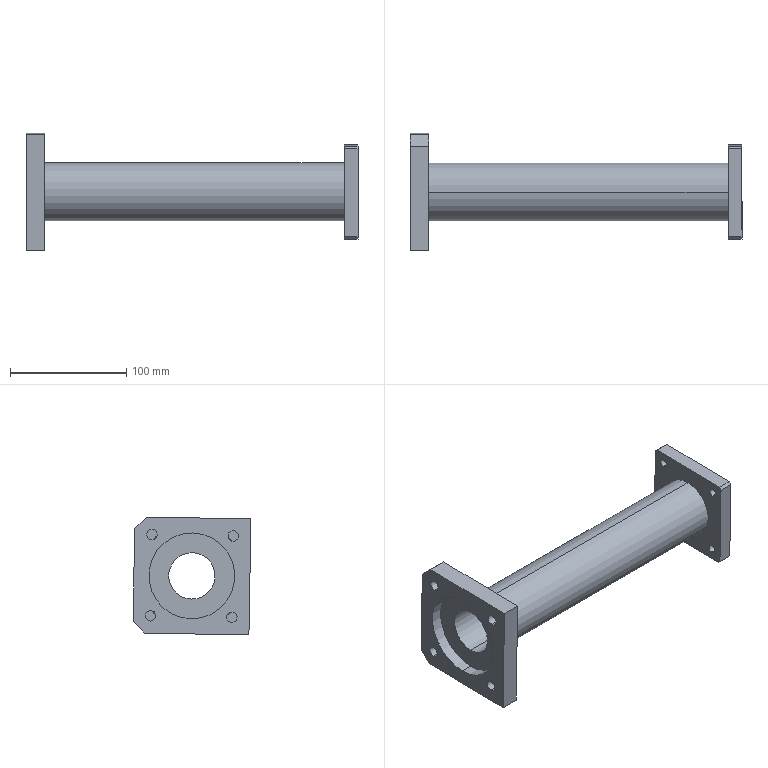Component | SolidWorks | CylinderSeat-1 | 1 solid | 41 faces | box 286 x 101.56 x 101.56 mm | volume 346031 mm3 | cylinder 22 | plane 19 | commonest cylinder face diameters 6.8 x8 9 x8 50 x2 40 x2 74 x2
build123d program:
from build123d import *

# Parameters (mm, degrees)
SKETCH1_W           = 100
SKETCH1_H           = 100
BOSS_EXTRUDE1_DEPTH = 16
SKETCH2_R           = 37
CUT_EXTRUDE1_DEPTH  = 10
SKETCH3_R           = 20
CUT_EXTRUDE2_DEPTH  = 72.414
SKETCH4_R           = 25
SKETCH4_R_2         = 20
BOSS_EXTRUDE2_DEPTH = 258
SKETCH5_W           = 80
SKETCH5_H           = 80
SKETCH5_R           = 20
BOSS_EXTRUDE3_DEPTH = 12
CHAMFER1_SIZE       = 10
SKETCH6_R           = 4.5
CUT_EXTRUDE3_DEPTH  = 20
SKETCH7_R           = 3.4
CUT_EXTRUDE4_DEPTH  = 20
CHAMFER2_SIZE       = 2


with BuildPart() as part:
    # Sketch1 → Boss-Extrude1 (new body)
    with BuildSketch(Plane.XY):
        Rectangle(SKETCH1_W, SKETCH1_H)
    extrude(amount=BOSS_EXTRUDE1_DEPTH)

    # Sketch2 → Cut-Extrude1 (cut)
    with BuildSketch(Plane.XY.offset(16)):
        Circle(SKETCH2_R)
    extrude(amount=-CUT_EXTRUDE1_DEPTH, mode=Mode.SUBTRACT)

    # Sketch3 → Cut-Extrude2 (cut, through all)
    with BuildSketch(Plane.XY.offset(6)):
        Circle(SKETCH3_R)
    extrude(amount=-CUT_EXTRUDE2_DEPTH, mode=Mode.SUBTRACT)

    # Sketch4 → Boss-Extrude2 (add)
    with BuildSketch(Plane(origin=(0, 0, 0), x_dir=(-1, 0, 0), z_dir=(0, 0, -1))):
        with Locations(Location((0, 0, 0), (0, 0, 180))):
            Circle(SKETCH4_R)
        with Locations(Location((0, 0, 0), (0, 0, 180))):
            Circle(SKETCH4_R_2, mode=Mode.SUBTRACT)
    extrude(amount=BOSS_EXTRUDE2_DEPTH)

    # Sketch5 → Boss-Extrude3 (add)
    with BuildSketch(Plane(origin=(0, 0, -258), x_dir=(-1, 0, 0), z_dir=(0, 0, -1))):
        Rectangle(SKETCH5_W, SKETCH5_H)
        with Locations(Location((0, 0, 0), (0, 0, 180))):
            Circle(SKETCH5_R, mode=Mode.SUBTRACT)
    extrude(amount=BOSS_EXTRUDE3_DEPTH)

    # Chamfer1
    chamfer1_edges = [part.edges().sort_by_distance(p)[0] for p in [
        (-50, 50, 8),
        (50, 50, 8),
    ]]
    chamfer(chamfer1_edges, length=CHAMFER1_SIZE)

    # Sketch6 → Cut-Extrude3 (cut)
    with BuildSketch(Plane.XY.offset(16)):
        with Locations((-35, 35)):
            Circle(SKETCH6_R)
        with Locations((35, 35)):
            Circle(SKETCH6_R)
        with Locations((35, -35)):
            Circle(SKETCH6_R)
        with Locations((-35, -35)):
            Circle(SKETCH6_R)
    extrude(amount=-CUT_EXTRUDE3_DEPTH, mode=Mode.SUBTRACT)

    # Sketch7 → Cut-Extrude4 (cut)
    with BuildSketch(Plane(origin=(0, 0, -270), x_dir=(-1, 0, 0), z_dir=(0, 0, -1))):
        with Locations((-30, 30)):
            Circle(SKETCH7_R)
        with Locations((30, 30)):
            Circle(SKETCH7_R)
        with Locations((30, -30)):
            Circle(SKETCH7_R)
        with Locations((-30, -30)):
            Circle(SKETCH7_R)
    extrude(amount=-CUT_EXTRUDE4_DEPTH, mode=Mode.SUBTRACT)

    # Chamfer2
    chamfer2_edges = [part.edges().sort_by_distance(p)[0] for p in [
        (-40, -40, -264),
        (-40, 40, -264),
        (40, 40, -264),
        (40, -40, -264),
    ]]
    chamfer(chamfer2_edges, length=CHAMFER2_SIZE)


solid = part.part

# Placed as in the assembly
solid = solid.moved(Location((683.004, 1299.706, 687.116), (1, -90, 0)))